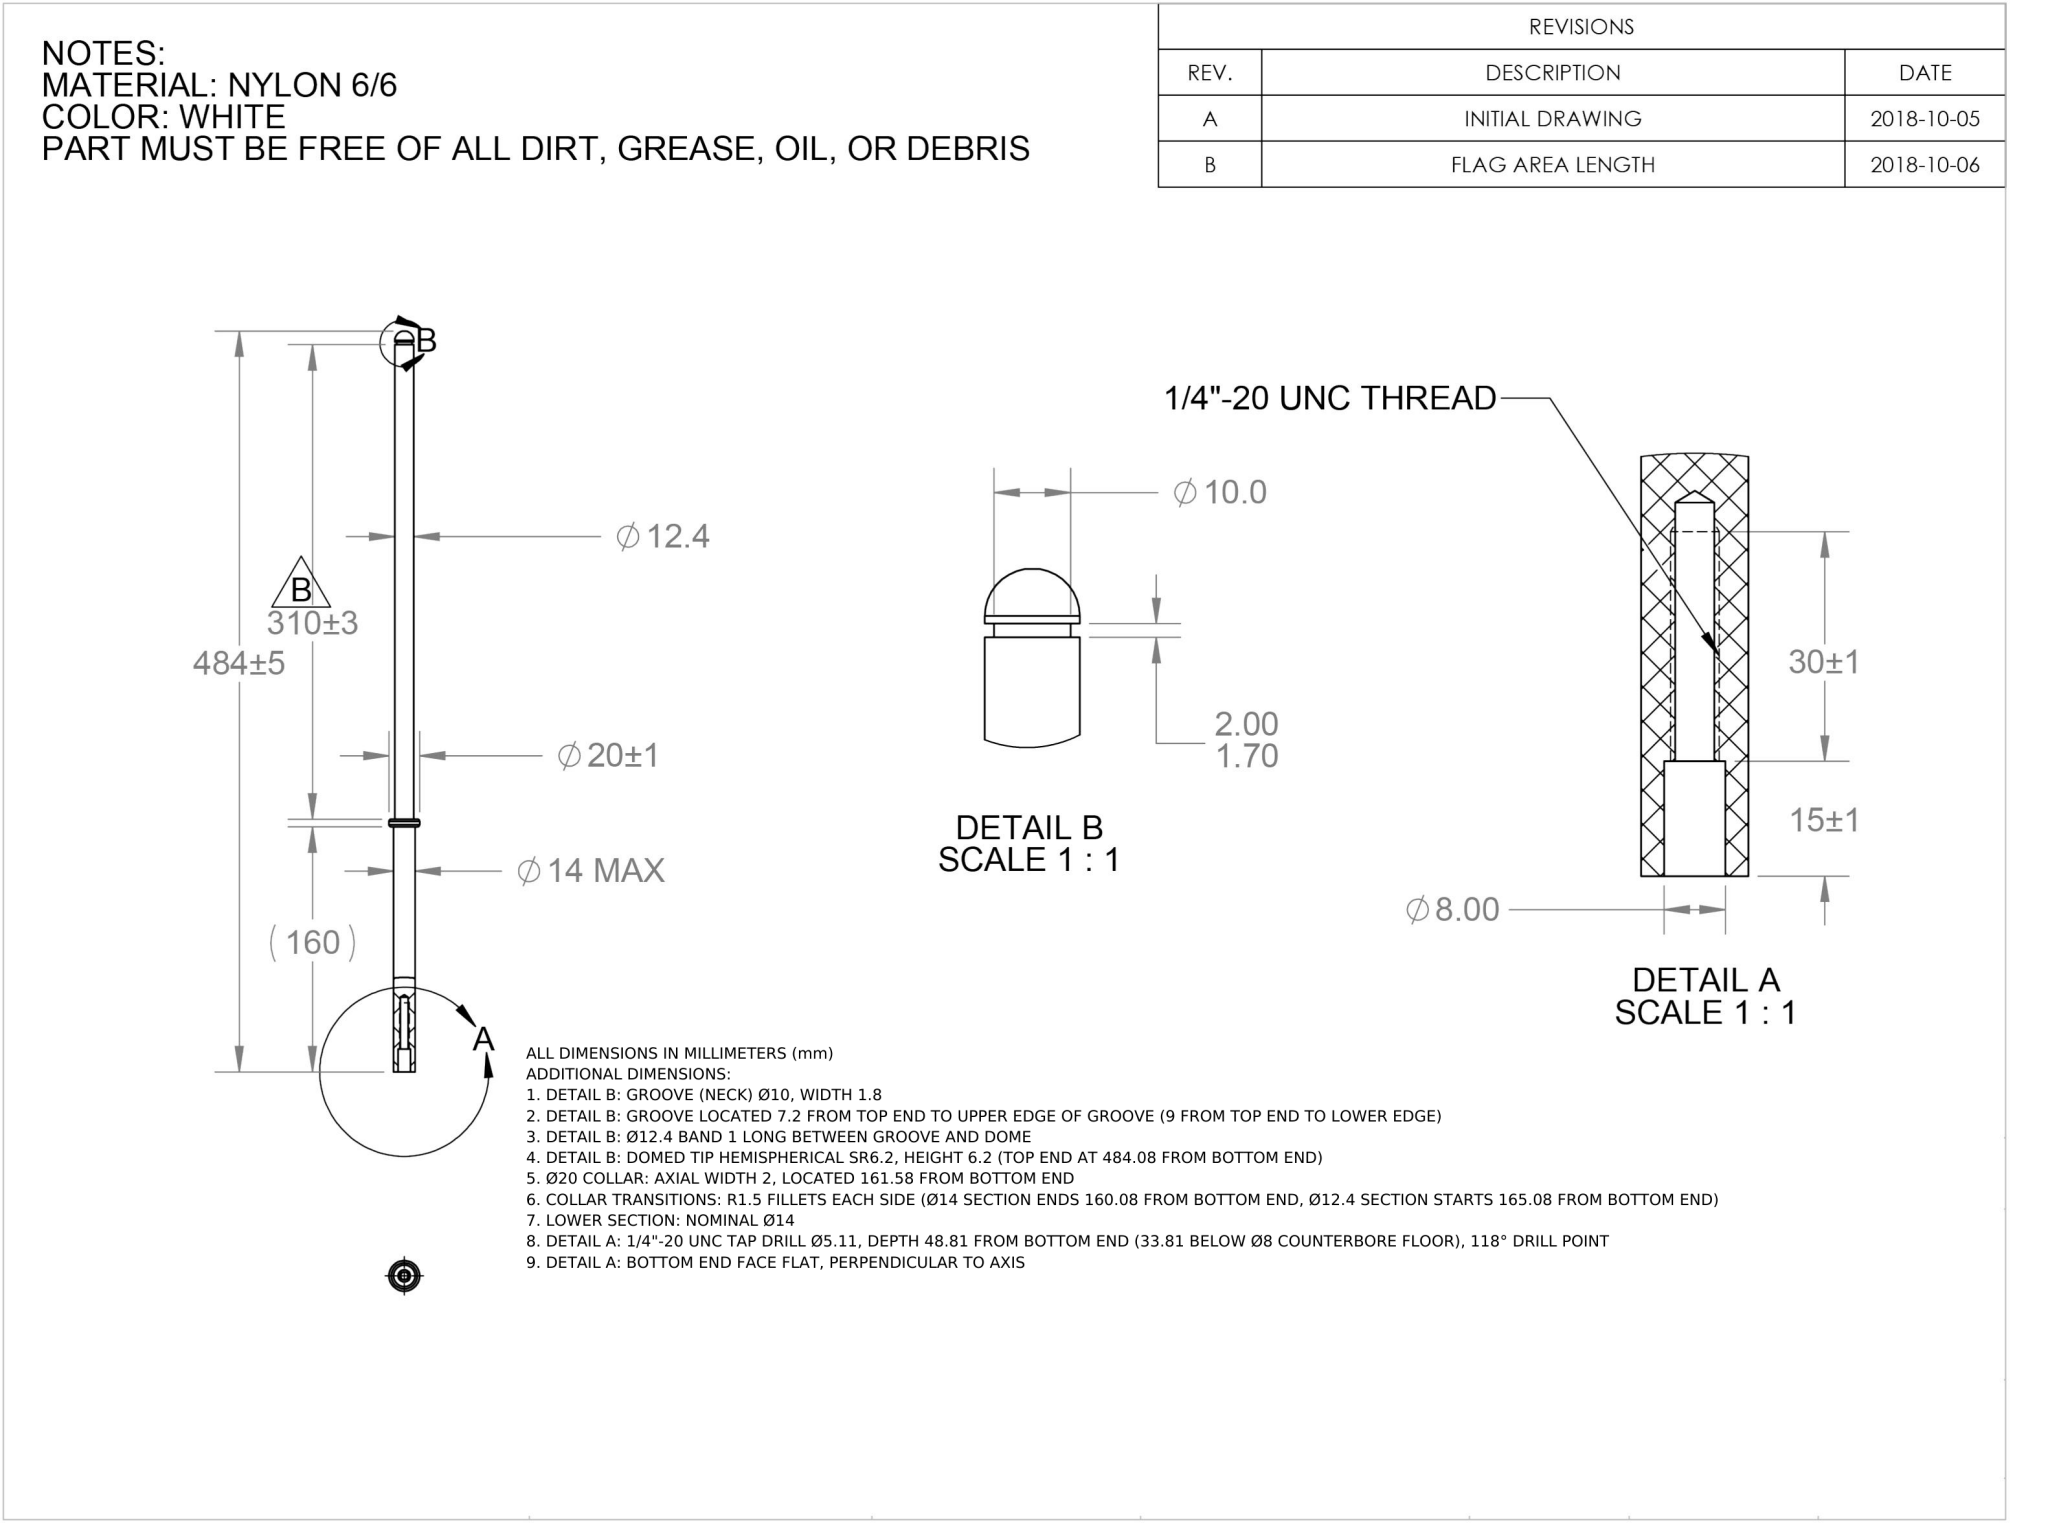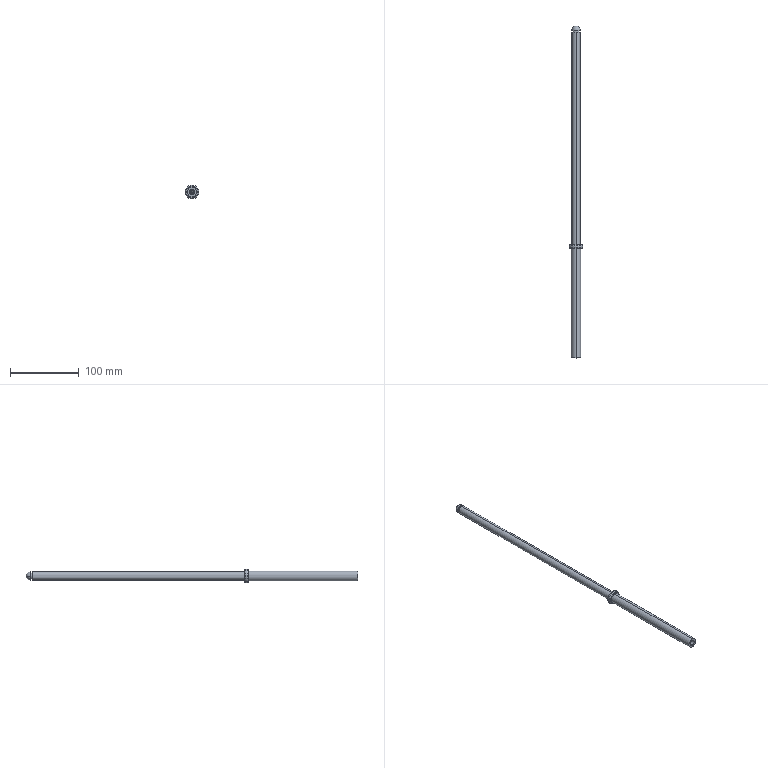Part | NX | mm | 1 solid | 29 faces | box 20 x 484 x 20 mm | volume 62896 mm3 | cylinder 14 | plane 7 | torus 4 | cone 2 | sphere 2 | commonest cylinder face diameters 12.4 x4 5.105 x2 8 x2 14 x2 20 x2 10 x2
STEP:
#1=COLOUR_RGB('',1.,1.,1.);
#2=FILL_AREA_STYLE_COLOUR('',#1);
#3=FILL_AREA_STYLE('',(#2));
#4=SURFACE_STYLE_FILL_AREA(#3);
#5=SURFACE_SIDE_STYLE('',(#4));
#6=SURFACE_STYLE_USAGE(.BOTH.,#5);
#7=PRESENTATION_STYLE_ASSIGNMENT((#6));
#8=CARTESIAN_POINT('',(0.,48.81,2.553));
#9=VERTEX_POINT('',#8);
#10=CARTESIAN_POINT('',(0.,15.,2.553));
#11=VERTEX_POINT('',#10);
#12=CARTESIAN_POINT('',(0.,15.,2.553));
#13=DIRECTION('',(0.,-1.,0.));
#14=VECTOR('',#13,1000.);
#15=LINE('',#12,#14);
#16=EDGE_CURVE('',#9,#11,#15,.T.);
#17=ORIENTED_EDGE('',*,*,#16,.F.);
#18=CARTESIAN_POINT('',(0.,48.81,-2.553));
#19=VERTEX_POINT('',#18);
#20=CARTESIAN_POINT('',(0.,48.81,0.));
#21=DIRECTION('',(0.,-1.,0.));
#22=DIRECTION('',(0.,0.,-1.));
#23=AXIS2_PLACEMENT_3D('',#20,#21,#22);
#24=CIRCLE('',#23,2.553);
#25=EDGE_CURVE('',#19,#9,#24,.T.);
#26=ORIENTED_EDGE('',*,*,#25,.F.);
#27=CARTESIAN_POINT('',(0.,15.,-2.553));
#28=VERTEX_POINT('',#27);
#29=CARTESIAN_POINT('',(0.,15.,-2.553));
#30=DIRECTION('',(0.,-1.,0.));
#31=VECTOR('',#30,1000.);
#32=LINE('',#29,#31);
#33=EDGE_CURVE('',#19,#28,#32,.T.);
#34=ORIENTED_EDGE('',*,*,#33,.T.);
#35=CARTESIAN_POINT('',(0.,15.,0.));
#36=DIRECTION('',(0.,-1.,0.));
#37=DIRECTION('',(0.,0.,-1.));
#38=AXIS2_PLACEMENT_3D('',#35,#36,#37);
#39=CIRCLE('',#38,2.553);
#40=EDGE_CURVE('',#28,#11,#39,.T.);
#41=ORIENTED_EDGE('',*,*,#40,.T.);
#42=EDGE_LOOP('',(#17,#26,#34,#41));
#43=FACE_OUTER_BOUND('',#42,.T.);
#44=CARTESIAN_POINT('',(0.,15.,0.));
#45=DIRECTION('',(0.,-1.,0.));
#46=DIRECTION('',(0.,0.,-1.));
#47=AXIS2_PLACEMENT_3D('',#44,#45,#46);
#48=CYLINDRICAL_SURFACE('',#47,2.553);
#49=ADVANCED_FACE('',(#43),#48,.F.);
#50=STYLED_ITEM('',(#7),#49);
#51=PRESENTATION_LAYER_ASSIGNMENT('','',(#50));
#52=(LENGTH_UNIT()NAMED_UNIT(*)SI_UNIT(.MILLI.,.METRE.));
#53=UNCERTAINTY_MEASURE_WITH_UNIT(LENGTH_MEASURE(0.00001),#52,'','');
#54=(NAMED_UNIT(*)PLANE_ANGLE_UNIT()SI_UNIT($,.RADIAN.));
#55=(NAMED_UNIT(*)SI_UNIT($,.STERADIAN.)SOLID_ANGLE_UNIT());
#56=(GEOMETRIC_REPRESENTATION_CONTEXT(3)GLOBAL_UNCERTAINTY_ASSIGNED_CONTEXT((#53))GLOBAL_UNIT_ASSIGNED_CONTEXT((#52,#54,#55))REPRESENTATION_CONTEXT('',''));
#57=MECHANICAL_DESIGN_GEOMETRIC_PRESENTATION_REPRESENTATION('',(#50),#56);
#58=COLOUR_RGB('',1.,1.,1.);
#59=FILL_AREA_STYLE_COLOUR('',#58);
#60=FILL_AREA_STYLE('',(#59));
#61=SURFACE_STYLE_FILL_AREA(#60);
#62=SURFACE_SIDE_STYLE('',(#61));
#63=SURFACE_STYLE_USAGE(.BOTH.,#62);
#64=PRESENTATION_STYLE_ASSIGNMENT((#63));
#65=CARTESIAN_POINT('',(0.,48.81,0.));
#66=DIRECTION('',(0.,-1.,0.));
#67=DIRECTION('',(0.,0.,-1.));
#68=AXIS2_PLACEMENT_3D('',#65,#66,#67);
#69=CIRCLE('',#68,2.553);
#70=EDGE_CURVE('',#9,#19,#69,.T.);
#71=ORIENTED_EDGE('',*,*,#70,.F.);
#72=ORIENTED_EDGE('',*,*,#16,.T.);
#73=CARTESIAN_POINT('',(0.,15.,0.));
#74=DIRECTION('',(0.,-1.,0.));
#75=DIRECTION('',(0.,0.,-1.));
#76=AXIS2_PLACEMENT_3D('',#73,#74,#75);
#77=CIRCLE('',#76,2.553);
#78=EDGE_CURVE('',#11,#28,#77,.T.);
#79=ORIENTED_EDGE('',*,*,#78,.T.);
#80=ORIENTED_EDGE('',*,*,#33,.F.);
#81=EDGE_LOOP('',(#71,#72,#79,#80));
#82=FACE_OUTER_BOUND('',#81,.T.);
#83=CARTESIAN_POINT('',(0.,15.,0.));
#84=DIRECTION('',(0.,-1.,0.));
#85=DIRECTION('',(0.,0.,-1.));
#86=AXIS2_PLACEMENT_3D('',#83,#84,#85);
#87=CYLINDRICAL_SURFACE('',#86,2.553);
#88=ADVANCED_FACE('',(#82),#87,.F.);
#89=STYLED_ITEM('',(#64),#88);
#90=PRESENTATION_LAYER_ASSIGNMENT('','',(#89));
#91=(LENGTH_UNIT()NAMED_UNIT(*)SI_UNIT(.MILLI.,.METRE.));
#92=UNCERTAINTY_MEASURE_WITH_UNIT(LENGTH_MEASURE(0.00001),#91,'','');
#93=(NAMED_UNIT(*)PLANE_ANGLE_UNIT()SI_UNIT($,.RADIAN.));
#94=(NAMED_UNIT(*)SI_UNIT($,.STERADIAN.)SOLID_ANGLE_UNIT());
#95=(GEOMETRIC_REPRESENTATION_CONTEXT(3)GLOBAL_UNCERTAINTY_ASSIGNED_CONTEXT((#92))GLOBAL_UNIT_ASSIGNED_CONTEXT((#91,#93,#94))REPRESENTATION_CONTEXT('',''));
#96=MECHANICAL_DESIGN_GEOMETRIC_PRESENTATION_REPRESENTATION('',(#89),#95);
#97=COLOUR_RGB('',1.,1.,1.);
#98=FILL_AREA_STYLE_COLOUR('',#97);
#99=FILL_AREA_STYLE('',(#98));
#100=SURFACE_STYLE_FILL_AREA(#99);
#101=SURFACE_SIDE_STYLE('',(#100));
#102=SURFACE_STYLE_USAGE(.BOTH.,#101);
#103=PRESENTATION_STYLE_ASSIGNMENT((#102));
#104=CARTESIAN_POINT('',(0.,163.581,-10.));
#105=VERTEX_POINT('',#104);
#106=CARTESIAN_POINT('',(0.,163.581,10.));
#107=VERTEX_POINT('',#106);
#108=CARTESIAN_POINT('',(0.,163.581,0.));
#109=DIRECTION('',(0.,-1.,0.));
#110=DIRECTION('',(0.,0.,1.));
#111=AXIS2_PLACEMENT_3D('',#108,#109,#110);
#112=CIRCLE('',#111,10.);
#113=EDGE_CURVE('',#105,#107,#112,.T.);
#114=ORIENTED_EDGE('',*,*,#113,.F.);
#115=CARTESIAN_POINT('',(0.,165.081,-8.5));
#116=VERTEX_POINT('',#115);
#117=CARTESIAN_POINT('',(0.,163.581,-8.5));
#118=DIRECTION('',(1.,0.,0.));
#119=DIRECTION('',(0.,0.,-1.));
#120=AXIS2_PLACEMENT_3D('',#117,#118,#119);
#121=CIRCLE('',#120,1.5);
#122=EDGE_CURVE('',#105,#116,#121,.T.);
#123=ORIENTED_EDGE('',*,*,#122,.T.);
#124=CARTESIAN_POINT('',(0.,165.081,8.5));
#125=VERTEX_POINT('',#124);
#126=CARTESIAN_POINT('',(0.,165.081,0.));
#127=DIRECTION('',(0.,1.,0.));
#128=DIRECTION('',(0.,0.,1.));
#129=AXIS2_PLACEMENT_3D('',#126,#127,#128);
#130=CIRCLE('',#129,8.5);
#131=EDGE_CURVE('',#125,#116,#130,.T.);
#132=ORIENTED_EDGE('',*,*,#131,.F.);
#133=CARTESIAN_POINT('',(0.,163.581,8.5));
#134=DIRECTION('',(-1.,0.,0.));
#135=DIRECTION('',(0.,0.,1.));
#136=AXIS2_PLACEMENT_3D('',#133,#134,#135);
#137=CIRCLE('',#136,1.5);
#138=EDGE_CURVE('',#107,#125,#137,.T.);
#139=ORIENTED_EDGE('',*,*,#138,.F.);
#140=EDGE_LOOP('',(#114,#123,#132,#139));
#141=FACE_OUTER_BOUND('',#140,.T.);
#142=CARTESIAN_POINT('',(0.,163.581,0.));
#143=DIRECTION('',(0.,1.,0.));
#144=DIRECTION('',(0.,0.,1.));
#145=AXIS2_PLACEMENT_3D('',#142,#143,#144);
#146=TOROIDAL_SURFACE('',#145,8.5,1.5);
#147=ADVANCED_FACE('',(#141),#146,.T.);
#148=CARTESIAN_POINT('',(0.,161.581,10.));
#149=VERTEX_POINT('',#148);
#150=CARTESIAN_POINT('',(0.,161.581,-10.));
#151=VERTEX_POINT('',#150);
#152=CARTESIAN_POINT('',(0.,161.581,0.));
#153=DIRECTION('',(0.,1.,0.));
#154=DIRECTION('',(0.,0.,-1.));
#155=AXIS2_PLACEMENT_3D('',#152,#153,#154);
#156=CIRCLE('',#155,10.);
#157=EDGE_CURVE('',#149,#151,#156,.T.);
#158=ORIENTED_EDGE('',*,*,#157,.F.);
#159=CARTESIAN_POINT('',(0.,160.081,8.5));
#160=VERTEX_POINT('',#159);
#161=CARTESIAN_POINT('',(0.,161.581,8.5));
#162=DIRECTION('',(1.,0.,-0.));
#163=DIRECTION('',(-0.,0.,-1.));
#164=AXIS2_PLACEMENT_3D('',#161,#162,#163);
#165=CIRCLE('',#164,1.5);
#166=EDGE_CURVE('',#149,#160,#165,.T.);
#167=ORIENTED_EDGE('',*,*,#166,.T.);
#168=CARTESIAN_POINT('',(0.,160.081,-8.5));
#169=VERTEX_POINT('',#168);
#170=CARTESIAN_POINT('',(0.,160.081,0.));
#171=DIRECTION('',(0.,-1.,0.));
#172=DIRECTION('',(0.,0.,-1.));
#173=AXIS2_PLACEMENT_3D('',#170,#171,#172);
#174=CIRCLE('',#173,8.5);
#175=EDGE_CURVE('',#169,#160,#174,.T.);
#176=ORIENTED_EDGE('',*,*,#175,.F.);
#177=CARTESIAN_POINT('',(0.,161.581,-8.5));
#178=DIRECTION('',(-1.,0.,0.));
#179=DIRECTION('',(0.,0.,1.));
#180=AXIS2_PLACEMENT_3D('',#177,#178,#179);
#181=CIRCLE('',#180,1.5);
#182=EDGE_CURVE('',#151,#169,#181,.T.);
#183=ORIENTED_EDGE('',*,*,#182,.F.);
#184=EDGE_LOOP('',(#158,#167,#176,#183));
#185=FACE_OUTER_BOUND('',#184,.T.);
#186=CARTESIAN_POINT('',(0.,161.581,0.));
#187=DIRECTION('',(0.,-1.,0.));
#188=DIRECTION('',(0.,0.,-1.));
#189=AXIS2_PLACEMENT_3D('',#186,#187,#188);
#190=TOROIDAL_SURFACE('',#189,8.5,1.5);
#191=ADVANCED_FACE('',(#185),#190,.T.);
#192=CARTESIAN_POINT('',(-0.,50.344,0.));
#193=VERTEX_POINT('',#192);
#194=CARTESIAN_POINT('',(0.,48.81,-2.553));
#195=DIRECTION('',(0.,-0.515,-0.8572));
#196=VECTOR('',#195,1000.);
#197=LINE('',#194,#196);
#198=EDGE_CURVE('',#193,#19,#197,.T.);
#199=ORIENTED_EDGE('',*,*,#198,.F.);
#200=CARTESIAN_POINT('',(0.,48.81,2.553));
#201=DIRECTION('',(0.,-0.515,0.8572));
#202=VECTOR('',#201,1000.);
#203=LINE('',#200,#202);
#204=EDGE_CURVE('',#193,#9,#203,.T.);
#205=ORIENTED_EDGE('',*,*,#204,.T.);
#206=ORIENTED_EDGE('',*,*,#70,.T.);
#207=EDGE_LOOP('',(#199,#205,#206));
#208=FACE_OUTER_BOUND('',#207,.T.);
#209=CARTESIAN_POINT('',(0.,48.81,0.));
#210=DIRECTION('',(0.,-1.,0.));
#211=DIRECTION('',(0.,0.,-1.));
#212=AXIS2_PLACEMENT_3D('',#209,#210,#211);
#213=CONICAL_SURFACE('',#212,2.553,1.03);
#214=ADVANCED_FACE('',(#208),#213,.F.);
#215=CARTESIAN_POINT('',(0.,0.,-4.));
#216=VERTEX_POINT('',#215);
#217=CARTESIAN_POINT('',(0.,0.,4.));
#218=VERTEX_POINT('',#217);
#219=CARTESIAN_POINT('',(0.,0.,0.));
#220=DIRECTION('',(0.,1.,0.));
#221=DIRECTION('',(0.,0.,1.));
#222=AXIS2_PLACEMENT_3D('',#219,#220,#221);
#223=CIRCLE('',#222,4.);
#224=EDGE_CURVE('',#216,#218,#223,.T.);
#225=ORIENTED_EDGE('',*,*,#224,.F.);
#226=CARTESIAN_POINT('',(0.,15.,-4.));
#227=VERTEX_POINT('',#226);
#228=CARTESIAN_POINT('',(0.,0.,-4.));
#229=DIRECTION('',(0.,1.,0.));
#230=VECTOR('',#229,1000.);
#231=LINE('',#228,#230);
#232=EDGE_CURVE('',#216,#227,#231,.T.);
#233=ORIENTED_EDGE('',*,*,#232,.T.);
#234=CARTESIAN_POINT('',(0.,15.,4.));
#235=VERTEX_POINT('',#234);
#236=CARTESIAN_POINT('',(0.,15.,0.));
#237=DIRECTION('',(0.,1.,0.));
#238=DIRECTION('',(0.,0.,1.));
#239=AXIS2_PLACEMENT_3D('',#236,#237,#238);
#240=CIRCLE('',#239,4.);
#241=EDGE_CURVE('',#227,#235,#240,.T.);
#242=ORIENTED_EDGE('',*,*,#241,.T.);
#243=CARTESIAN_POINT('',(0.,0.,4.));
#244=DIRECTION('',(0.,1.,0.));
#245=VECTOR('',#244,1000.);
#246=LINE('',#243,#245);
#247=EDGE_CURVE('',#218,#235,#246,.T.);
#248=ORIENTED_EDGE('',*,*,#247,.F.);
#249=EDGE_LOOP('',(#225,#233,#242,#248));
#250=FACE_OUTER_BOUND('',#249,.T.);
#251=CARTESIAN_POINT('',(0.,0.,0.));
#252=DIRECTION('',(0.,1.,0.));
#253=DIRECTION('',(0.,0.,1.));
#254=AXIS2_PLACEMENT_3D('',#251,#252,#253);
#255=CYLINDRICAL_SURFACE('',#254,4.);
#256=ADVANCED_FACE('',(#250),#255,.F.);
#257=CARTESIAN_POINT('',(0.,0.,7.));
#258=VERTEX_POINT('',#257);
#259=CARTESIAN_POINT('',(0.,0.,-7.));
#260=VERTEX_POINT('',#259);
#261=CARTESIAN_POINT('',(0.,0.,0.));
#262=DIRECTION('',(0.,1.,0.));
#263=DIRECTION('',(0.,0.,1.));
#264=AXIS2_PLACEMENT_3D('',#261,#262,#263);
#265=CIRCLE('',#264,7.);
#266=EDGE_CURVE('',#258,#260,#265,.T.);
#267=ORIENTED_EDGE('',*,*,#266,.T.);
#268=CARTESIAN_POINT('',(0.,160.081,-7.));
#269=VERTEX_POINT('',#268);
#270=CARTESIAN_POINT('',(0.,0.,-7.));
#271=DIRECTION('',(0.,1.,0.));
#272=VECTOR('',#271,1000.);
#273=LINE('',#270,#272);
#274=EDGE_CURVE('',#260,#269,#273,.T.);
#275=ORIENTED_EDGE('',*,*,#274,.T.);
#276=CARTESIAN_POINT('',(0.,160.081,7.));
#277=VERTEX_POINT('',#276);
#278=CARTESIAN_POINT('',(0.,160.081,0.));
#279=DIRECTION('',(0.,1.,0.));
#280=DIRECTION('',(0.,0.,1.));
#281=AXIS2_PLACEMENT_3D('',#278,#279,#280);
#282=CIRCLE('',#281,7.);
#283=EDGE_CURVE('',#277,#269,#282,.T.);
#284=ORIENTED_EDGE('',*,*,#283,.F.);
#285=CARTESIAN_POINT('',(0.,0.,7.));
#286=DIRECTION('',(0.,1.,0.));
#287=VECTOR('',#286,1000.);
#288=LINE('',#285,#287);
#289=EDGE_CURVE('',#258,#277,#288,.T.);
#290=ORIENTED_EDGE('',*,*,#289,.F.);
#291=EDGE_LOOP('',(#267,#275,#284,#290));
#292=FACE_OUTER_BOUND('',#291,.T.);
#293=CARTESIAN_POINT('',(0.,0.,0.));
#294=DIRECTION('',(0.,1.,0.));
#295=DIRECTION('',(0.,0.,1.));
#296=AXIS2_PLACEMENT_3D('',#293,#294,#295);
#297=CYLINDRICAL_SURFACE('',#296,7.);
#298=ADVANCED_FACE('',(#292),#297,.T.);
#299=ORIENTED_EDGE('',*,*,#157,.T.);
#300=CARTESIAN_POINT('',(0.,0.,-10.));
#301=DIRECTION('',(0.,1.,0.));
#302=VECTOR('',#301,1000.);
#303=LINE('',#300,#302);
#304=EDGE_CURVE('',#151,#105,#303,.T.);
#305=ORIENTED_EDGE('',*,*,#304,.T.);
#306=ORIENTED_EDGE('',*,*,#113,.T.);
#307=CARTESIAN_POINT('',(0.,0.,10.));
#308=DIRECTION('',(0.,1.,0.));
#309=VECTOR('',#308,1000.);
#310=LINE('',#307,#309);
#311=EDGE_CURVE('',#149,#107,#310,.T.);
#312=ORIENTED_EDGE('',*,*,#311,.F.);
#313=EDGE_LOOP('',(#299,#305,#306,#312));
#314=FACE_OUTER_BOUND('',#313,.T.);
#315=CARTESIAN_POINT('',(0.,0.,0.));
#316=DIRECTION('',(0.,1.,0.));
#317=DIRECTION('',(0.,0.,1.));
#318=AXIS2_PLACEMENT_3D('',#315,#316,#317);
#319=CYLINDRICAL_SURFACE('',#318,10.);
#320=ADVANCED_FACE('',(#314),#319,.T.);
#321=CARTESIAN_POINT('',(0.,165.081,6.2));
#322=VERTEX_POINT('',#321);
#323=CARTESIAN_POINT('',(0.,165.081,-6.2));
#324=VERTEX_POINT('',#323);
#325=CARTESIAN_POINT('',(0.,165.081,0.));
#326=DIRECTION('',(0.,1.,0.));
#327=DIRECTION('',(0.,0.,1.));
#328=AXIS2_PLACEMENT_3D('',#325,#326,#327);
#329=CIRCLE('',#328,6.2);
#330=EDGE_CURVE('',#322,#324,#329,.T.);
#331=ORIENTED_EDGE('',*,*,#330,.T.);
#332=CARTESIAN_POINT('',(0.,475.081,-6.2));
#333=VERTEX_POINT('',#332);
#334=CARTESIAN_POINT('',(0.,0.,-6.2));
#335=DIRECTION('',(0.,1.,0.));
#336=VECTOR('',#335,1000.);
#337=LINE('',#334,#336);
#338=EDGE_CURVE('',#324,#333,#337,.T.);
#339=ORIENTED_EDGE('',*,*,#338,.T.);
#340=CARTESIAN_POINT('',(0.,475.081,6.2));
#341=VERTEX_POINT('',#340);
#342=CARTESIAN_POINT('',(0.,475.081,0.));
#343=DIRECTION('',(0.,1.,0.));
#344=DIRECTION('',(0.,0.,1.));
#345=AXIS2_PLACEMENT_3D('',#342,#343,#344);
#346=CIRCLE('',#345,6.2);
#347=EDGE_CURVE('',#341,#333,#346,.T.);
#348=ORIENTED_EDGE('',*,*,#347,.F.);
#349=CARTESIAN_POINT('',(0.,0.,6.2));
#350=DIRECTION('',(0.,1.,0.));
#351=VECTOR('',#350,1000.);
#352=LINE('',#349,#351);
#353=EDGE_CURVE('',#322,#341,#352,.T.);
#354=ORIENTED_EDGE('',*,*,#353,.F.);
#355=EDGE_LOOP('',(#331,#339,#348,#354));
#356=FACE_OUTER_BOUND('',#355,.T.);
#357=CARTESIAN_POINT('',(0.,0.,0.));
#358=DIRECTION('',(0.,1.,0.));
#359=DIRECTION('',(0.,0.,1.));
#360=AXIS2_PLACEMENT_3D('',#357,#358,#359);
#361=CYLINDRICAL_SURFACE('',#360,6.2);
#362=ADVANCED_FACE('',(#356),#361,.T.);
#363=CARTESIAN_POINT('',(0.,475.081,5.));
#364=VERTEX_POINT('',#363);
#365=CARTESIAN_POINT('',(0.,475.081,-5.));
#366=VERTEX_POINT('',#365);
#367=CARTESIAN_POINT('',(0.,475.081,0.));
#368=DIRECTION('',(0.,1.,0.));
#369=DIRECTION('',(0.,0.,1.));
#370=AXIS2_PLACEMENT_3D('',#367,#368,#369);
#371=CIRCLE('',#370,5.);
#372=EDGE_CURVE('',#364,#366,#371,.T.);
#373=ORIENTED_EDGE('',*,*,#372,.T.);
#374=CARTESIAN_POINT('',(0.,476.881,-5.));
#375=VERTEX_POINT('',#374);
#376=CARTESIAN_POINT('',(0.,0.,-5.));
#377=DIRECTION('',(0.,1.,0.));
#378=VECTOR('',#377,1000.);
#379=LINE('',#376,#378);
#380=EDGE_CURVE('',#366,#375,#379,.T.);
#381=ORIENTED_EDGE('',*,*,#380,.T.);
#382=CARTESIAN_POINT('',(0.,476.881,5.));
#383=VERTEX_POINT('',#382);
#384=CARTESIAN_POINT('',(0.,476.881,0.));
#385=DIRECTION('',(0.,1.,0.));
#386=DIRECTION('',(0.,0.,1.));
#387=AXIS2_PLACEMENT_3D('',#384,#385,#386);
#388=CIRCLE('',#387,5.);
#389=EDGE_CURVE('',#383,#375,#388,.T.);
#390=ORIENTED_EDGE('',*,*,#389,.F.);
#391=CARTESIAN_POINT('',(0.,0.,5.));
#392=DIRECTION('',(0.,1.,0.));
#393=VECTOR('',#392,1000.);
#394=LINE('',#391,#393);
#395=EDGE_CURVE('',#364,#383,#394,.T.);
#396=ORIENTED_EDGE('',*,*,#395,.F.);
#397=EDGE_LOOP('',(#373,#381,#390,#396));
#398=FACE_OUTER_BOUND('',#397,.T.);
#399=CARTESIAN_POINT('',(0.,0.,0.));
#400=DIRECTION('',(0.,1.,0.));
#401=DIRECTION('',(0.,0.,1.));
#402=AXIS2_PLACEMENT_3D('',#399,#400,#401);
#403=CYLINDRICAL_SURFACE('',#402,5.);
#404=ADVANCED_FACE('',(#398),#403,.T.);
#405=CARTESIAN_POINT('',(0.,476.881,6.2));
#406=VERTEX_POINT('',#405);
#407=CARTESIAN_POINT('',(0.,476.881,-6.2));
#408=VERTEX_POINT('',#407);
#409=CARTESIAN_POINT('',(0.,476.881,0.));
#410=DIRECTION('',(0.,1.,0.));
#411=DIRECTION('',(0.,0.,1.));
#412=AXIS2_PLACEMENT_3D('',#409,#410,#411);
#413=CIRCLE('',#412,6.2);
#414=EDGE_CURVE('',#406,#408,#413,.T.);
#415=ORIENTED_EDGE('',*,*,#414,.T.);
#416=CARTESIAN_POINT('',(0.,477.881,-6.2));
#417=VERTEX_POINT('',#416);
#418=CARTESIAN_POINT('',(0.,0.,-6.2));
#419=DIRECTION('',(0.,1.,0.));
#420=VECTOR('',#419,1000.);
#421=LINE('',#418,#420);
#422=EDGE_CURVE('',#408,#417,#421,.T.);
#423=ORIENTED_EDGE('',*,*,#422,.T.);
#424=CARTESIAN_POINT('',(6.2,477.881,0.));
#425=VERTEX_POINT('',#424);
#426=CARTESIAN_POINT('',(0.,477.881,0.));
#427=DIRECTION('',(0.,1.,0.));
#428=DIRECTION('',(0.,0.,1.));
#429=AXIS2_PLACEMENT_3D('',#426,#427,#428);
#430=CIRCLE('',#429,6.2);
#431=EDGE_CURVE('',#425,#417,#430,.T.);
#432=ORIENTED_EDGE('',*,*,#431,.F.);
#433=CARTESIAN_POINT('',(0.,477.881,6.2));
#434=VERTEX_POINT('',#433);
#435=CARTESIAN_POINT('',(0.,477.881,0.));
#436=DIRECTION('',(0.,1.,0.));
#437=DIRECTION('',(0.,0.,1.));
#438=AXIS2_PLACEMENT_3D('',#435,#436,#437);
#439=CIRCLE('',#438,6.2);
#440=EDGE_CURVE('',#434,#425,#439,.T.);
#441=ORIENTED_EDGE('',*,*,#440,.F.);
#442=CARTESIAN_POINT('',(0.,0.,6.2));
#443=DIRECTION('',(0.,1.,0.));
#444=VECTOR('',#443,1000.);
#445=LINE('',#442,#444);
#446=EDGE_CURVE('',#406,#434,#445,.T.);
#447=ORIENTED_EDGE('',*,*,#446,.F.);
#448=EDGE_LOOP('',(#415,#423,#432,#441,#447));
#449=FACE_OUTER_BOUND('',#448,.T.);
#450=CARTESIAN_POINT('',(0.,0.,0.));
#451=DIRECTION('',(0.,1.,0.));
#452=DIRECTION('',(0.,0.,1.));
#453=AXIS2_PLACEMENT_3D('',#450,#451,#452);
#454=CYLINDRICAL_SURFACE('',#453,6.2);
#455=ADVANCED_FACE('',(#449),#454,.T.);
#456=CARTESIAN_POINT('',(-6.2,477.881,0.));
#457=VERTEX_POINT('',#456);
#458=CARTESIAN_POINT('',(0.,477.881,0.));
#459=DIRECTION('',(0.,1.,0.));
#460=DIRECTION('',(0.,0.,1.));
#461=AXIS2_PLACEMENT_3D('',#458,#459,#460);
#462=CIRCLE('',#461,6.2);
#463=EDGE_CURVE('',#457,#434,#462,.T.);
#464=ORIENTED_EDGE('',*,*,#463,.T.);
#465=ORIENTED_EDGE('',*,*,#440,.T.);
#466=CARTESIAN_POINT('',(1.,484.,0.));
#467=VERTEX_POINT('',#466);
#468=CARTESIAN_POINT('',(0.,477.881,0.));
#469=DIRECTION('',(-0.,0.,1.));
#470=DIRECTION('',(1.,0.,0.));
#471=AXIS2_PLACEMENT_3D('',#468,#469,#470);
#472=CIRCLE('',#471,6.2);
#473=EDGE_CURVE('',#425,#467,#472,.T.);
#474=ORIENTED_EDGE('',*,*,#473,.T.);
#475=CARTESIAN_POINT('',(-1.,484.,0.));
#476=VERTEX_POINT('',#475);
#477=CARTESIAN_POINT('',(0.,484.,0.));
#478=DIRECTION('',(0.,1.,0.));
#479=DIRECTION('',(0.,0.,1.));
#480=AXIS2_PLACEMENT_3D('',#477,#478,#479);
#481=CIRCLE('',#480,1.);
#482=EDGE_CURVE('',#476,#467,#481,.T.);
#483=ORIENTED_EDGE('',*,*,#482,.F.);
#484=CARTESIAN_POINT('',(0.,477.881,0.));
#485=DIRECTION('',(0.,0.,-1.));
#486=DIRECTION('',(-1.,0.,0.));
#487=AXIS2_PLACEMENT_3D('',#484,#485,#486);
#488=CIRCLE('',#487,6.2);
#489=EDGE_CURVE('',#457,#476,#488,.T.);
#490=ORIENTED_EDGE('',*,*,#489,.F.);
#491=EDGE_LOOP('',(#464,#465,#474,#483,#490));
#492=FACE_OUTER_BOUND('',#491,.T.);
#493=CARTESIAN_POINT('',(0.,477.881,0.));
#494=DIRECTION('',(0.,0.,1.));
#495=DIRECTION('',(-1.,0.,0.));
#496=AXIS2_PLACEMENT_3D('',#493,#494,#495);
#497=SPHERICAL_SURFACE('',#496,6.2);
#498=ADVANCED_FACE('',(#492),#497,.T.);
#499=ORIENTED_EDGE('',*,*,#482,.T.);
#500=CARTESIAN_POINT('',(0.,484.,0.));
#501=DIRECTION('',(0.,1.,0.));
#502=DIRECTION('',(0.,0.,1.));
#503=AXIS2_PLACEMENT_3D('',#500,#501,#502);
#504=CIRCLE('',#503,1.);
#505=EDGE_CURVE('',#467,#476,#504,.T.);
#506=ORIENTED_EDGE('',*,*,#505,.T.);
#507=EDGE_LOOP('',(#499,#506));
#508=FACE_OUTER_BOUND('',#507,.T.);
#509=CARTESIAN_POINT('',(0.,484.,0.));
#510=DIRECTION('',(0.,1.,0.));
#511=DIRECTION('',(0.,0.,1.));
#512=AXIS2_PLACEMENT_3D('',#509,#510,#511);
#513=PLANE('',#512);
#514=ADVANCED_FACE('',(#508),#513,.T.);
#515=ORIENTED_EDGE('',*,*,#473,.F.);
#516=ORIENTED_EDGE('',*,*,#431,.T.);
#517=CARTESIAN_POINT('',(0.,477.881,0.));
#518=DIRECTION('',(0.,1.,0.));
#519=DIRECTION('',(0.,0.,1.));
#520=AXIS2_PLACEMENT_3D('',#517,#518,#519);
#521=CIRCLE('',#520,6.2);
#522=EDGE_CURVE('',#417,#457,#521,.T.);
#523=ORIENTED_EDGE('',*,*,#522,.T.);
#524=ORIENTED_EDGE('',*,*,#489,.T.);
#525=ORIENTED_EDGE('',*,*,#505,.F.);
#526=EDGE_LOOP('',(#515,#516,#523,#524,#525));
#527=FACE_OUTER_BOUND('',#526,.T.);
#528=CARTESIAN_POINT('',(0.,477.881,0.));
#529=DIRECTION('',(0.,0.,1.));
#530=DIRECTION('',(-1.,0.,0.));
#531=AXIS2_PLACEMENT_3D('',#528,#529,#530);
#532=SPHERICAL_SURFACE('',#531,6.2);
#533=ADVANCED_FACE('',(#527),#532,.T.);
#534=ORIENTED_EDGE('',*,*,#422,.F.);
#535=CARTESIAN_POINT('',(0.,476.881,0.));
#536=DIRECTION('',(0.,1.,0.));
#537=DIRECTION('',(0.,0.,1.));
#538=AXIS2_PLACEMENT_3D('',#535,#536,#537);
#539=CIRCLE('',#538,6.2);
#540=EDGE_CURVE('',#408,#406,#539,.T.);
#541=ORIENTED_EDGE('',*,*,#540,.T.);
#542=ORIENTED_EDGE('',*,*,#446,.T.);
#543=ORIENTED_EDGE('',*,*,#463,.F.);
#544=ORIENTED_EDGE('',*,*,#522,.F.);
#545=EDGE_LOOP('',(#534,#541,#542,#543,#544));
#546=FACE_OUTER_BOUND('',#545,.T.);
#547=CARTESIAN_POINT('',(0.,0.,0.));
#548=DIRECTION('',(0.,1.,0.));
#549=DIRECTION('',(0.,0.,1.));
#550=AXIS2_PLACEMENT_3D('',#547,#548,#549);
#551=CYLINDRICAL_SURFACE('',#550,6.2);
#552=ADVANCED_FACE('',(#546),#551,.T.);
#553=ORIENTED_EDGE('',*,*,#389,.T.);
#554=CARTESIAN_POINT('',(0.,476.881,0.));
#555=DIRECTION('',(0.,1.,0.));
#556=DIRECTION('',(0.,0.,1.));
#557=AXIS2_PLACEMENT_3D('',#554,#555,#556);
#558=CIRCLE('',#557,5.);
#559=EDGE_CURVE('',#375,#383,#558,.T.);
#560=ORIENTED_EDGE('',*,*,#559,.T.);
#561=EDGE_LOOP('',(#553,#560));
#562=FACE_BOUND('',#561,.T.);
#563=ORIENTED_EDGE('',*,*,#414,.F.);
#564=ORIENTED_EDGE('',*,*,#540,.F.);
#565=EDGE_LOOP('',(#563,#564));
#566=FACE_OUTER_BOUND('',#565,.T.);
#567=CARTESIAN_POINT('',(-5.,476.881,0.));
#568=DIRECTION('',(0.,-1.,0.));
#569=DIRECTION('',(0.,0.,-1.));
#570=AXIS2_PLACEMENT_3D('',#567,#568,#569);
#571=PLANE('',#570);
#572=ADVANCED_FACE('',(#562,#566),#571,.T.);
#573=ORIENTED_EDGE('',*,*,#380,.F.);
#574=CARTESIAN_POINT('',(0.,475.081,0.));
#575=DIRECTION('',(0.,1.,0.));
#576=DIRECTION('',(0.,0.,1.));
#577=AXIS2_PLACEMENT_3D('',#574,#575,#576);
#578=CIRCLE('',#577,5.);
#579=EDGE_CURVE('',#366,#364,#578,.T.);
#580=ORIENTED_EDGE('',*,*,#579,.T.);
#581=ORIENTED_EDGE('',*,*,#395,.T.);
#582=ORIENTED_EDGE('',*,*,#559,.F.);
#583=EDGE_LOOP('',(#573,#580,#581,#582));
#584=FACE_OUTER_BOUND('',#583,.T.);
#585=CARTESIAN_POINT('',(0.,0.,0.));
#586=DIRECTION('',(0.,1.,0.));
#587=DIRECTION('',(0.,0.,1.));
#588=AXIS2_PLACEMENT_3D('',#585,#586,#587);
#589=CYLINDRICAL_SURFACE('',#588,5.);
#590=ADVANCED_FACE('',(#584),#589,.T.);
#591=ORIENTED_EDGE('',*,*,#347,.T.);
#592=CARTESIAN_POINT('',(0.,475.081,0.));
#593=DIRECTION('',(0.,1.,0.));
#594=DIRECTION('',(0.,0.,1.));
#595=AXIS2_PLACEMENT_3D('',#592,#593,#594);
#596=CIRCLE('',#595,6.2);
#597=EDGE_CURVE('',#333,#341,#596,.T.);
#598=ORIENTED_EDGE('',*,*,#597,.T.);
#599=EDGE_LOOP('',(#591,#598));
#600=FACE_OUTER_BOUND('',#599,.T.);
#601=ORIENTED_EDGE('',*,*,#372,.F.);
#602=ORIENTED_EDGE('',*,*,#579,.F.);
#603=EDGE_LOOP('',(#601,#602));
#604=FACE_BOUND('',#603,.T.);
#605=CARTESIAN_POINT('',(-5.,475.081,0.));
#606=DIRECTION('',(0.,1.,0.));
#607=DIRECTION('',(0.,0.,1.));
#608=AXIS2_PLACEMENT_3D('',#605,#606,#607);
#609=PLANE('',#608);
#610=ADVANCED_FACE('',(#600,#604),#609,.T.);
#611=ORIENTED_EDGE('',*,*,#338,.F.);
#612=CARTESIAN_POINT('',(0.,165.081,0.));
#613=DIRECTION('',(0.,1.,0.));
#614=DIRECTION('',(0.,0.,1.));
#615=AXIS2_PLACEMENT_3D('',#612,#613,#614);
#616=CIRCLE('',#615,6.2);
#617=EDGE_CURVE('',#324,#322,#616,.T.);
#618=ORIENTED_EDGE('',*,*,#617,.T.);
#619=ORIENTED_EDGE('',*,*,#353,.T.);
#620=ORIENTED_EDGE('',*,*,#597,.F.);
#621=EDGE_LOOP('',(#611,#618,#619,#620));
#622=FACE_OUTER_BOUND('',#621,.T.);
#623=CARTESIAN_POINT('',(0.,0.,0.));
#624=DIRECTION('',(0.,1.,0.));
#625=DIRECTION('',(0.,0.,1.));
#626=AXIS2_PLACEMENT_3D('',#623,#624,#625);
#627=CYLINDRICAL_SURFACE('',#626,6.2);
#628=ADVANCED_FACE('',(#622),#627,.T.);
#629=ORIENTED_EDGE('',*,*,#131,.T.);
#630=CARTESIAN_POINT('',(0.,165.081,0.));
#631=DIRECTION('',(0.,1.,0.));
#632=DIRECTION('',(0.,0.,1.));
#633=AXIS2_PLACEMENT_3D('',#630,#631,#632);
#634=CIRCLE('',#633,8.5);
#635=EDGE_CURVE('',#116,#125,#634,.T.);
#636=ORIENTED_EDGE('',*,*,#635,.T.);
#637=EDGE_LOOP('',(#629,#636));
#638=FACE_OUTER_BOUND('',#637,.T.);
#639=ORIENTED_EDGE('',*,*,#330,.F.);
#640=ORIENTED_EDGE('',*,*,#617,.F.);
#641=EDGE_LOOP('',(#639,#640));
#642=FACE_BOUND('',#641,.T.);
#643=CARTESIAN_POINT('',(-6.2,165.081,0.));
#644=DIRECTION('',(0.,1.,0.));
#645=DIRECTION('',(0.,0.,1.));
#646=AXIS2_PLACEMENT_3D('',#643,#644,#645);
#647=PLANE('',#646);
#648=ADVANCED_FACE('',(#638,#642),#647,.T.);
#649=ORIENTED_EDGE('',*,*,#304,.F.);
#650=CARTESIAN_POINT('',(0.,161.581,0.));
#651=DIRECTION('',(0.,1.,0.));
#652=DIRECTION('',(0.,0.,-1.));
#653=AXIS2_PLACEMENT_3D('',#650,#651,#652);
#654=CIRCLE('',#653,10.);
#655=EDGE_CURVE('',#151,#149,#654,.T.);
#656=ORIENTED_EDGE('',*,*,#655,.T.);
#657=ORIENTED_EDGE('',*,*,#311,.T.);
#658=CARTESIAN_POINT('',(0.,163.581,0.));
#659=DIRECTION('',(0.,-1.,0.));
#660=DIRECTION('',(0.,0.,1.));
#661=AXIS2_PLACEMENT_3D('',#658,#659,#660);
#662=CIRCLE('',#661,10.);
#663=EDGE_CURVE('',#107,#105,#662,.T.);
#664=ORIENTED_EDGE('',*,*,#663,.T.);
#665=EDGE_LOOP('',(#649,#656,#657,#664));
#666=FACE_OUTER_BOUND('',#665,.T.);
#667=CARTESIAN_POINT('',(0.,0.,0.));
#668=DIRECTION('',(0.,1.,0.));
#669=DIRECTION('',(0.,0.,1.));
#670=AXIS2_PLACEMENT_3D('',#667,#668,#669);
#671=CYLINDRICAL_SURFACE('',#670,10.);
#672=ADVANCED_FACE('',(#666),#671,.T.);
#673=ORIENTED_EDGE('',*,*,#175,.T.);
#674=CARTESIAN_POINT('',(0.,160.081,0.));
#675=DIRECTION('',(0.,-1.,0.));
#676=DIRECTION('',(0.,0.,-1.));
#677=AXIS2_PLACEMENT_3D('',#674,#675,#676);
#678=CIRCLE('',#677,8.5);
#679=EDGE_CURVE('',#160,#169,#678,.T.);
#680=ORIENTED_EDGE('',*,*,#679,.T.);
#681=EDGE_LOOP('',(#673,#680));
#682=FACE_OUTER_BOUND('',#681,.T.);
#683=ORIENTED_EDGE('',*,*,#283,.T.);
#684=CARTESIAN_POINT('',(0.,160.081,0.));
#685=DIRECTION('',(0.,1.,0.));
#686=DIRECTION('',(0.,0.,1.));
#687=AXIS2_PLACEMENT_3D('',#684,#685,#686);
#688=CIRCLE('',#687,7.);
#689=EDGE_CURVE('',#269,#277,#688,.T.);
#690=ORIENTED_EDGE('',*,*,#689,.T.);
#691=EDGE_LOOP('',(#683,#690));
#692=FACE_BOUND('',#691,.T.);
#693=CARTESIAN_POINT('',(-10.,160.081,0.));
#694=DIRECTION('',(0.,-1.,0.));
#695=DIRECTION('',(0.,0.,-1.));
#696=AXIS2_PLACEMENT_3D('',#693,#694,#695);
#697=PLANE('',#696);
#698=ADVANCED_FACE('',(#682,#692),#697,.T.);
#699=ORIENTED_EDGE('',*,*,#274,.F.);
#700=CARTESIAN_POINT('',(0.,0.,0.));
#701=DIRECTION('',(0.,1.,0.));
#702=DIRECTION('',(0.,0.,1.));
#703=AXIS2_PLACEMENT_3D('',#700,#701,#702);
#704=CIRCLE('',#703,7.);
#705=EDGE_CURVE('',#260,#258,#704,.T.);
#706=ORIENTED_EDGE('',*,*,#705,.T.);
#707=ORIENTED_EDGE('',*,*,#289,.T.);
#708=ORIENTED_EDGE('',*,*,#689,.F.);
#709=EDGE_LOOP('',(#699,#706,#707,#708));
#710=FACE_OUTER_BOUND('',#709,.T.);
#711=CARTESIAN_POINT('',(0.,0.,0.));
#712=DIRECTION('',(0.,1.,0.));
#713=DIRECTION('',(0.,0.,1.));
#714=AXIS2_PLACEMENT_3D('',#711,#712,#713);
#715=CYLINDRICAL_SURFACE('',#714,7.);
#716=ADVANCED_FACE('',(#710),#715,.T.);
#717=CARTESIAN_POINT('',(0.,0.,0.));
#718=DIRECTION('',(0.,1.,0.));
#719=DIRECTION('',(0.,0.,1.));
#720=AXIS2_PLACEMENT_3D('',#717,#718,#719);
#721=CIRCLE('',#720,4.);
#722=EDGE_CURVE('',#218,#216,#721,.T.);
#723=ORIENTED_EDGE('',*,*,#722,.T.);
#724=ORIENTED_EDGE('',*,*,#224,.T.);
#725=EDGE_LOOP('',(#723,#724));
#726=FACE_BOUND('',#725,.T.);
#727=ORIENTED_EDGE('',*,*,#266,.F.);
#728=ORIENTED_EDGE('',*,*,#705,.F.);
#729=EDGE_LOOP('',(#727,#728));
#730=FACE_OUTER_BOUND('',#729,.T.);
#731=CARTESIAN_POINT('',(-7.,0.,0.));
#732=DIRECTION('',(0.,-1.,0.));
#733=DIRECTION('',(0.,0.,-1.));
#734=AXIS2_PLACEMENT_3D('',#731,#732,#733);
#735=PLANE('',#734);
#736=ADVANCED_FACE('',(#726,#730),#735,.T.);
#737=ORIENTED_EDGE('',*,*,#232,.F.);
#738=ORIENTED_EDGE('',*,*,#722,.F.);
#739=ORIENTED_EDGE('',*,*,#247,.T.);
#740=CARTESIAN_POINT('',(0.,15.,0.));
#741=DIRECTION('',(0.,1.,0.));
#742=DIRECTION('',(0.,0.,1.));
#743=AXIS2_PLACEMENT_3D('',#740,#741,#742);
#744=CIRCLE('',#743,4.);
#745=EDGE_CURVE('',#235,#227,#744,.T.);
#746=ORIENTED_EDGE('',*,*,#745,.T.);
#747=EDGE_LOOP('',(#737,#738,#739,#746));
#748=FACE_OUTER_BOUND('',#747,.T.);
#749=CARTESIAN_POINT('',(0.,0.,0.));
#750=DIRECTION('',(0.,1.,0.));
#751=DIRECTION('',(0.,0.,1.));
#752=AXIS2_PLACEMENT_3D('',#749,#750,#751);
#753=CYLINDRICAL_SURFACE('',#752,4.);
#754=ADVANCED_FACE('',(#748),#753,.F.);
#755=ORIENTED_EDGE('',*,*,#40,.F.);
#756=ORIENTED_EDGE('',*,*,#78,.F.);
#757=EDGE_LOOP('',(#755,#756));
#758=FACE_BOUND('',#757,.T.);
#759=ORIENTED_EDGE('',*,*,#745,.F.);
#760=ORIENTED_EDGE('',*,*,#241,.F.);
#761=EDGE_LOOP('',(#759,#760));
#762=FACE_OUTER_BOUND('',#761,.T.);
#763=CARTESIAN_POINT('',(-4.,15.,0.));
#764=DIRECTION('',(0.,-1.,0.));
#765=DIRECTION('',(0.,0.,-1.));
#766=AXIS2_PLACEMENT_3D('',#763,#764,#765);
#767=PLANE('',#766);
#768=ADVANCED_FACE('',(#758,#762),#767,.T.);
#769=ORIENTED_EDGE('',*,*,#204,.F.);
#770=ORIENTED_EDGE('',*,*,#198,.T.);
#771=ORIENTED_EDGE('',*,*,#25,.T.);
#772=EDGE_LOOP('',(#769,#770,#771));
#773=FACE_OUTER_BOUND('',#772,.T.);
#774=CARTESIAN_POINT('',(0.,48.81,0.));
#775=DIRECTION('',(0.,-1.,0.));
#776=DIRECTION('',(0.,0.,-1.));
#777=AXIS2_PLACEMENT_3D('',#774,#775,#776);
#778=CONICAL_SURFACE('',#777,2.553,1.03);
#779=ADVANCED_FACE('',(#773),#778,.F.);
#780=ORIENTED_EDGE('',*,*,#166,.F.);
#781=ORIENTED_EDGE('',*,*,#655,.F.);
#782=ORIENTED_EDGE('',*,*,#182,.T.);
#783=ORIENTED_EDGE('',*,*,#679,.F.);
#784=EDGE_LOOP('',(#780,#781,#782,#783));
#785=FACE_OUTER_BOUND('',#784,.T.);
#786=CARTESIAN_POINT('',(0.,161.581,0.));
#787=DIRECTION('',(0.,-1.,0.));
#788=DIRECTION('',(0.,0.,-1.));
#789=AXIS2_PLACEMENT_3D('',#786,#787,#788);
#790=TOROIDAL_SURFACE('',#789,8.5,1.5);
#791=ADVANCED_FACE('',(#785),#790,.T.);
#792=ORIENTED_EDGE('',*,*,#122,.F.);
#793=ORIENTED_EDGE('',*,*,#663,.F.);
#794=ORIENTED_EDGE('',*,*,#138,.T.);
#795=ORIENTED_EDGE('',*,*,#635,.F.);
#796=EDGE_LOOP('',(#792,#793,#794,#795));
#797=FACE_OUTER_BOUND('',#796,.T.);
#798=CARTESIAN_POINT('',(0.,163.581,0.));
#799=DIRECTION('',(0.,1.,0.));
#800=DIRECTION('',(0.,0.,1.));
#801=AXIS2_PLACEMENT_3D('',#798,#799,#800);
#802=TOROIDAL_SURFACE('',#801,8.5,1.5);
#803=ADVANCED_FACE('',(#797),#802,.T.);
#804=CLOSED_SHELL('',(#147,#191,#88,#214,#256,#298,#320,#362,#404,#455,#498,#514,#533,#552,#572,#590,#610,#628,#648,#672,#698,#716,#736,#754,#768,#779,#49,#791,#803));
#805=MANIFOLD_SOLID_BREP('',#804);
#806=STYLED_ITEM('',(#103),#805);
#807=PRESENTATION_LAYER_ASSIGNMENT('','',(#806));
#808=(LENGTH_UNIT()NAMED_UNIT(*)SI_UNIT(.MILLI.,.METRE.));
#809=UNCERTAINTY_MEASURE_WITH_UNIT(LENGTH_MEASURE(0.00001),#808,'','');
#810=(NAMED_UNIT(*)PLANE_ANGLE_UNIT()SI_UNIT($,.RADIAN.));
#811=(NAMED_UNIT(*)SI_UNIT($,.STERADIAN.)SOLID_ANGLE_UNIT());
#812=(GEOMETRIC_REPRESENTATION_CONTEXT(3)GLOBAL_UNCERTAINTY_ASSIGNED_CONTEXT((#809))GLOBAL_UNIT_ASSIGNED_CONTEXT((#808,#810,#811))REPRESENTATION_CONTEXT('',''));
#813=MECHANICAL_DESIGN_GEOMETRIC_PRESENTATION_REPRESENTATION('',(#806),#812);
#814=COLOUR_RGB('',1.,1.,1.);
#815=FILL_AREA_STYLE_COLOUR('',#814);
#816=FILL_AREA_STYLE('',(#815));
#817=SURFACE_STYLE_FILL_AREA(#816);
#818=SURFACE_SIDE_STYLE('',(#817));
#819=SURFACE_STYLE_USAGE(.BOTH.,#818);
#820=PRESENTATION_STYLE_ASSIGNMENT((#819));
#821=CARTESIAN_POINT('',(0.,0.,0.));
#822=DIRECTION('',(0.,0.,1.));
#823=DIRECTION('',(1.,0.,0.));
#824=AXIS2_PLACEMENT_3D('',#821,#822,#823);
#825=(LENGTH_UNIT()NAMED_UNIT(*)SI_UNIT(.MILLI.,.METRE.));
#826=UNCERTAINTY_MEASURE_WITH_UNIT(LENGTH_MEASURE(0.00001),#825,'','');
#827=(NAMED_UNIT(*)PLANE_ANGLE_UNIT()SI_UNIT($,.RADIAN.));
#828=(NAMED_UNIT(*)SI_UNIT($,.STERADIAN.)SOLID_ANGLE_UNIT());
#829=(GEOMETRIC_REPRESENTATION_CONTEXT(3)GLOBAL_UNCERTAINTY_ASSIGNED_CONTEXT((#826))GLOBAL_UNIT_ASSIGNED_CONTEXT((#825,#827,#828))REPRESENTATION_CONTEXT('',''));
#830=ADVANCED_BREP_SHAPE_REPRESENTATION('',(#805,#824),#829);
#831=STYLED_ITEM('',(#820),#830);
#832=PRESENTATION_LAYER_ASSIGNMENT('','',(#831));
#833=(LENGTH_UNIT()NAMED_UNIT(*)SI_UNIT(.MILLI.,.METRE.));
#834=UNCERTAINTY_MEASURE_WITH_UNIT(LENGTH_MEASURE(0.00001),#833,'','');
#835=(NAMED_UNIT(*)PLANE_ANGLE_UNIT()SI_UNIT($,.RADIAN.));
#836=(NAMED_UNIT(*)SI_UNIT($,.STERADIAN.)SOLID_ANGLE_UNIT());
#837=(GEOMETRIC_REPRESENTATION_CONTEXT(3)GLOBAL_UNCERTAINTY_ASSIGNED_CONTEXT((#834))GLOBAL_UNIT_ASSIGNED_CONTEXT((#833,#835,#836))REPRESENTATION_CONTEXT('',''));
#838=MECHANICAL_DESIGN_GEOMETRIC_PRESENTATION_REPRESENTATION('',(#831),#837);